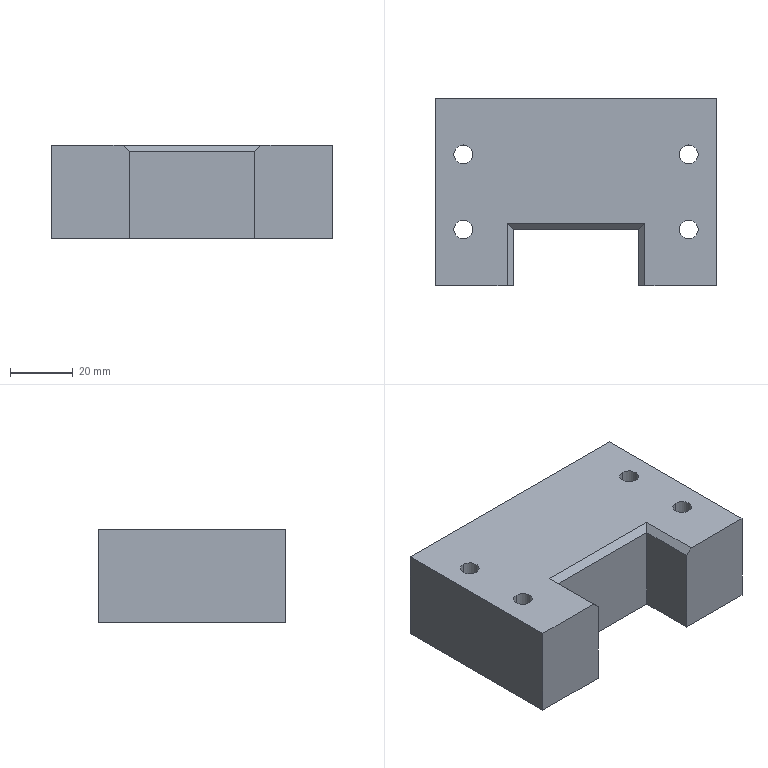Component | SolidWorks | JQ-2-0-006-1 | 1 solid | 29 faces | box 90 x 60 x 30 mm | volume 136495 mm3 | plane 13 | cylinder 12 | cone 4 | commonest cylinder face diameters 6 x8 4.2 x4
build123d program:
from build123d import *

# Parameters (mm, degrees)
SKETCH1_W             = 90
SKETCH1_H             = 30
BOSS_EXTRUDE1_DEPTH   = 60
M5_TAPPED_HOLE1_D     = 4.2
M5_TAPPED_HOLE1_DEPTH = 12.4
M5_TAPPED_HOLE1_TIP   = 1.262
SKETCH5_R             = 3
CUT_EXTRUDE3_DEPTH    = 60
SKETCH6_W             = 40
SKETCH6_H             = 30
CUT_EXTRUDE4_DEPTH    = 18
CHAMFER3_SIZE         = 2


with BuildPart() as part:
    # Sketch1 → Boss-Extrude1 (new body)
    with BuildSketch(Plane.XY):
        with Locations((45, 15)):
            Rectangle(SKETCH1_W, SKETCH1_H)
    extrude(amount=BOSS_EXTRUDE1_DEPTH)

    # M5 Tapped Hole1
    with Locations(Plane(origin=(0, 30, 0), x_dir=(-1, 0, 0), z_dir=(0, 1, 0))):
        with Locations((-25, 30), (-65, 30)):
            Hole(M5_TAPPED_HOLE1_D / 2, depth=M5_TAPPED_HOLE1_DEPTH)
            with Locations((0, 0, -(M5_TAPPED_HOLE1_DEPTH + M5_TAPPED_HOLE1_TIP / 2))):  # 118° drill point
                Cone(0, M5_TAPPED_HOLE1_D / 2, M5_TAPPED_HOLE1_TIP, mode=Mode.SUBTRACT)

    # Sketch5 → Cut-Extrude3 (cut)
    with BuildSketch(Plane(origin=(0, 30, 0), x_dir=(1, 0, 0), z_dir=(0, 1, 0))):
        with Locations(Location((9, -42, 0), (0, 0, 270))):
            Circle(SKETCH5_R)
        with Locations(Location((81, -42, 0), (0, 0, 270))):
            Circle(SKETCH5_R)
        with Locations(Location((81, -18, 0), (0, 0, 270))):
            Circle(SKETCH5_R)
        with Locations(Location((9, -18, 0), (0, 0, 270))):
            Circle(SKETCH5_R)
    extrude(amount=-CUT_EXTRUDE3_DEPTH, mode=Mode.SUBTRACT)

    # Sketch6 → Cut-Extrude4 (cut)
    with BuildSketch(Plane(origin=(0, 0, 0), x_dir=(-1, 0, 0), z_dir=(0, 0, -1))):
        with Locations((-45, 15)):
            Rectangle(SKETCH6_W, SKETCH6_H)
    extrude(amount=-CUT_EXTRUDE4_DEPTH, mode=Mode.SUBTRACT)

    # Chamfer3
    chamfer3_edges = [part.edges().sort_by_distance(p)[0] for p in [
        (45, 0, 18),
        (25, 0, 9),
        (65, 0, 9),
    ]]
    chamfer(chamfer3_edges, length=CHAMFER3_SIZE)


solid = part.part

# Placed as in the assembly
solid = solid.moved(Location((-307.058, -0.6609, 14.131), (-90, 0, 0)))
STEP:
#1=COLOUR_RGB('',0.7922,0.8196,0.9333);
#2=FILL_AREA_STYLE_COLOUR('',#1);
#3=FILL_AREA_STYLE('',(#2));
#4=SURFACE_STYLE_FILL_AREA(#3);
#5=SURFACE_SIDE_STYLE('',(#4));
#6=SURFACE_STYLE_USAGE(.BOTH.,#5);
#7=PRESENTATION_STYLE_ASSIGNMENT((#6));
#8=CARTESIAN_POINT('',(-11.735,0.5645,0.5563));
#9=VERTEX_POINT('',#8);
#10=CARTESIAN_POINT('',(-11.735,0.8008,0.5563));
#11=VERTEX_POINT('',#10);
#12=CARTESIAN_POINT('',(-11.735,0.6826,0.5563));
#13=DIRECTION('',(-0.,0.,-1.));
#14=DIRECTION('',(0.,1.,0.));
#15=AXIS2_PLACEMENT_3D('',#12,#13,#14);
#16=CIRCLE('',#15,0.1181);
#17=EDGE_CURVE('',#9,#11,#16,.T.);
#18=ORIENTED_EDGE('',*,*,#17,.F.);
#19=CARTESIAN_POINT('',(-11.735,0.5645,-0.6248));
#20=VERTEX_POINT('',#19);
#21=CARTESIAN_POINT('',(-11.735,0.5645,1.737));
#22=DIRECTION('',(-0.,0.,-1.));
#23=VECTOR('',#22,39.37);
#24=LINE('',#21,#23);
#25=EDGE_CURVE('',#9,#20,#24,.T.);
#26=ORIENTED_EDGE('',*,*,#25,.T.);
#27=CARTESIAN_POINT('',(-11.735,0.8008,-0.6248));
#28=VERTEX_POINT('',#27);
#29=CARTESIAN_POINT('',(-11.735,0.6826,-0.6248));
#30=DIRECTION('',(-0.,0.,-1.));
#31=DIRECTION('',(0.,1.,0.));
#32=AXIS2_PLACEMENT_3D('',#29,#30,#31);
#33=CIRCLE('',#32,0.1181);
#34=EDGE_CURVE('',#20,#28,#33,.T.);
#35=ORIENTED_EDGE('',*,*,#34,.T.);
#36=CARTESIAN_POINT('',(-11.735,0.8008,1.737));
#37=DIRECTION('',(-0.,0.,-1.));
#38=VECTOR('',#37,39.37);
#39=LINE('',#36,#38);
#40=EDGE_CURVE('',#11,#28,#39,.T.);
#41=ORIENTED_EDGE('',*,*,#40,.F.);
#42=EDGE_LOOP('',(#18,#26,#35,#41));
#43=FACE_OUTER_BOUND('',#42,.T.);
#44=CARTESIAN_POINT('',(-11.735,0.6826,1.737));
#45=DIRECTION('',(-0.,0.,-1.));
#46=DIRECTION('',(0.,1.,0.));
#47=AXIS2_PLACEMENT_3D('',#44,#45,#46);
#48=CYLINDRICAL_SURFACE('',#47,0.1181);
#49=ADVANCED_FACE('',(#43),#48,.F.);
#50=CARTESIAN_POINT('',(-8.9,0.5645,0.5563));
#51=VERTEX_POINT('',#50);
#52=CARTESIAN_POINT('',(-8.9,0.8008,0.5563));
#53=VERTEX_POINT('',#52);
#54=CARTESIAN_POINT('',(-8.9,0.6826,0.5563));
#55=DIRECTION('',(-0.,0.,-1.));
#56=DIRECTION('',(0.,1.,0.));
#57=AXIS2_PLACEMENT_3D('',#54,#55,#56);
#58=CIRCLE('',#57,0.1181);
#59=EDGE_CURVE('',#51,#53,#58,.T.);
#60=ORIENTED_EDGE('',*,*,#59,.F.);
#61=CARTESIAN_POINT('',(-8.9,0.5645,-0.6248));
#62=VERTEX_POINT('',#61);
#63=CARTESIAN_POINT('',(-8.9,0.5645,1.737));
#64=DIRECTION('',(-0.,0.,-1.));
#65=VECTOR('',#64,39.37);
#66=LINE('',#63,#65);
#67=EDGE_CURVE('',#51,#62,#66,.T.);
#68=ORIENTED_EDGE('',*,*,#67,.T.);
#69=CARTESIAN_POINT('',(-8.9,0.8008,-0.6248));
#70=VERTEX_POINT('',#69);
#71=CARTESIAN_POINT('',(-8.9,0.6826,-0.6248));
#72=DIRECTION('',(-0.,0.,-1.));
#73=DIRECTION('',(0.,1.,0.));
#74=AXIS2_PLACEMENT_3D('',#71,#72,#73);
#75=CIRCLE('',#74,0.1181);
#76=EDGE_CURVE('',#62,#70,#75,.T.);
#77=ORIENTED_EDGE('',*,*,#76,.T.);
#78=CARTESIAN_POINT('',(-8.9,0.8008,1.737));
#79=DIRECTION('',(-0.,0.,-1.));
#80=VECTOR('',#79,39.37);
#81=LINE('',#78,#80);
#82=EDGE_CURVE('',#53,#70,#81,.T.);
#83=ORIENTED_EDGE('',*,*,#82,.F.);
#84=EDGE_LOOP('',(#60,#68,#77,#83));
#85=FACE_OUTER_BOUND('',#84,.T.);
#86=CARTESIAN_POINT('',(-8.9,0.6826,1.737));
#87=DIRECTION('',(-0.,0.,-1.));
#88=DIRECTION('',(0.,1.,0.));
#89=AXIS2_PLACEMENT_3D('',#86,#87,#88);
#90=CYLINDRICAL_SURFACE('',#89,0.1181);
#91=ADVANCED_FACE('',(#85),#90,.F.);
#92=CARTESIAN_POINT('',(-8.9,1.509,0.5563));
#93=VERTEX_POINT('',#92);
#94=CARTESIAN_POINT('',(-8.9,1.746,0.5563));
#95=VERTEX_POINT('',#94);
#96=CARTESIAN_POINT('',(-8.9,1.628,0.5563));
#97=DIRECTION('',(-0.,0.,-1.));
#98=DIRECTION('',(0.,1.,0.));
#99=AXIS2_PLACEMENT_3D('',#96,#97,#98);
#100=CIRCLE('',#99,0.1181);
#101=EDGE_CURVE('',#93,#95,#100,.T.);
#102=ORIENTED_EDGE('',*,*,#101,.F.);
#103=CARTESIAN_POINT('',(-8.9,1.509,-0.6248));
#104=VERTEX_POINT('',#103);
#105=CARTESIAN_POINT('',(-8.9,1.509,1.737));
#106=DIRECTION('',(-0.,0.,-1.));
#107=VECTOR('',#106,39.37);
#108=LINE('',#105,#107);
#109=EDGE_CURVE('',#93,#104,#108,.T.);
#110=ORIENTED_EDGE('',*,*,#109,.T.);
#111=CARTESIAN_POINT('',(-8.9,1.746,-0.6248));
#112=VERTEX_POINT('',#111);
#113=CARTESIAN_POINT('',(-8.9,1.628,-0.6248));
#114=DIRECTION('',(-0.,0.,-1.));
#115=DIRECTION('',(0.,1.,0.));
#116=AXIS2_PLACEMENT_3D('',#113,#114,#115);
#117=CIRCLE('',#116,0.1181);
#118=EDGE_CURVE('',#104,#112,#117,.T.);
#119=ORIENTED_EDGE('',*,*,#118,.T.);
#120=CARTESIAN_POINT('',(-8.9,1.746,1.737));
#121=DIRECTION('',(-0.,0.,-1.));
#122=VECTOR('',#121,39.37);
#123=LINE('',#120,#122);
#124=EDGE_CURVE('',#95,#112,#123,.T.);
#125=ORIENTED_EDGE('',*,*,#124,.F.);
#126=EDGE_LOOP('',(#102,#110,#119,#125));
#127=FACE_OUTER_BOUND('',#126,.T.);
#128=CARTESIAN_POINT('',(-8.9,1.628,1.737));
#129=DIRECTION('',(-0.,0.,-1.));
#130=DIRECTION('',(0.,1.,0.));
#131=AXIS2_PLACEMENT_3D('',#128,#129,#130);
#132=CYLINDRICAL_SURFACE('',#131,0.1181);
#133=ADVANCED_FACE('',(#127),#132,.F.);
#134=CARTESIAN_POINT('',(-11.735,1.509,0.5563));
#135=VERTEX_POINT('',#134);
#136=CARTESIAN_POINT('',(-11.735,1.746,0.5563));
#137=VERTEX_POINT('',#136);
#138=CARTESIAN_POINT('',(-11.735,1.628,0.5563));
#139=DIRECTION('',(-0.,0.,-1.));
#140=DIRECTION('',(0.,1.,0.));
#141=AXIS2_PLACEMENT_3D('',#138,#139,#140);
#142=CIRCLE('',#141,0.1181);
#143=EDGE_CURVE('',#135,#137,#142,.T.);
#144=ORIENTED_EDGE('',*,*,#143,.F.);
#145=CARTESIAN_POINT('',(-11.735,1.509,-0.6248));
#146=VERTEX_POINT('',#145);
#147=CARTESIAN_POINT('',(-11.735,1.509,1.737));
#148=DIRECTION('',(-0.,0.,-1.));
#149=VECTOR('',#148,39.37);
#150=LINE('',#147,#149);
#151=EDGE_CURVE('',#135,#146,#150,.T.);
#152=ORIENTED_EDGE('',*,*,#151,.T.);
#153=CARTESIAN_POINT('',(-11.735,1.746,-0.6248));
#154=VERTEX_POINT('',#153);
#155=CARTESIAN_POINT('',(-11.735,1.628,-0.6248));
#156=DIRECTION('',(-0.,0.,-1.));
#157=DIRECTION('',(0.,1.,0.));
#158=AXIS2_PLACEMENT_3D('',#155,#156,#157);
#159=CIRCLE('',#158,0.1181);
#160=EDGE_CURVE('',#146,#154,#159,.T.);
#161=ORIENTED_EDGE('',*,*,#160,.T.);
#162=CARTESIAN_POINT('',(-11.735,1.746,1.737));
#163=DIRECTION('',(-0.,0.,-1.));
#164=VECTOR('',#163,39.37);
#165=LINE('',#162,#164);
#166=EDGE_CURVE('',#137,#154,#165,.T.);
#167=ORIENTED_EDGE('',*,*,#166,.F.);
#168=EDGE_LOOP('',(#144,#152,#161,#167));
#169=FACE_OUTER_BOUND('',#168,.T.);
#170=CARTESIAN_POINT('',(-11.735,1.628,1.737));
#171=DIRECTION('',(-0.,0.,-1.));
#172=DIRECTION('',(0.,1.,0.));
#173=AXIS2_PLACEMENT_3D('',#170,#171,#172);
#174=CYLINDRICAL_SURFACE('',#173,0.1181);
#175=ADVANCED_FACE('',(#169),#174,.F.);
#176=CARTESIAN_POINT('',(-11.105,1.072,-0.1366));
#177=VERTEX_POINT('',#176);
#178=CARTESIAN_POINT('',(-11.105,1.238,-0.1366));
#179=VERTEX_POINT('',#178);
#180=CARTESIAN_POINT('',(-11.105,1.155,-0.1366));
#181=DIRECTION('',(-0.,0.,-1.));
#182=DIRECTION('',(0.,1.,0.));
#183=AXIS2_PLACEMENT_3D('',#180,#181,#182);
#184=CIRCLE('',#183,0.08268);
#185=EDGE_CURVE('',#177,#179,#184,.T.);
#186=ORIENTED_EDGE('',*,*,#185,.F.);
#187=CARTESIAN_POINT('',(-11.105,1.072,-0.6248));
#188=VERTEX_POINT('',#187);
#189=CARTESIAN_POINT('',(-11.105,1.072,-0.6248));
#190=DIRECTION('',(-0.,0.,-1.));
#191=VECTOR('',#190,39.37);
#192=LINE('',#189,#191);
#193=EDGE_CURVE('',#177,#188,#192,.T.);
#194=ORIENTED_EDGE('',*,*,#193,.T.);
#195=CARTESIAN_POINT('',(-11.105,1.238,-0.6248));
#196=VERTEX_POINT('',#195);
#197=CARTESIAN_POINT('',(-11.105,1.155,-0.6248));
#198=DIRECTION('',(-0.,0.,-1.));
#199=DIRECTION('',(0.,1.,0.));
#200=AXIS2_PLACEMENT_3D('',#197,#198,#199);
#201=CIRCLE('',#200,0.08268);
#202=EDGE_CURVE('',#188,#196,#201,.T.);
#203=ORIENTED_EDGE('',*,*,#202,.T.);
#204=CARTESIAN_POINT('',(-11.105,1.238,-0.6248));
#205=DIRECTION('',(-0.,0.,-1.));
#206=VECTOR('',#205,39.37);
#207=LINE('',#204,#206);
#208=EDGE_CURVE('',#179,#196,#207,.T.);
#209=ORIENTED_EDGE('',*,*,#208,.F.);
#210=EDGE_LOOP('',(#186,#194,#203,#209));
#211=FACE_OUTER_BOUND('',#210,.T.);
#212=CARTESIAN_POINT('',(-11.105,1.155,-0.6248));
#213=DIRECTION('',(-0.,0.,-1.));
#214=DIRECTION('',(0.,1.,0.));
#215=AXIS2_PLACEMENT_3D('',#212,#213,#214);
#216=CYLINDRICAL_SURFACE('',#215,0.08268);
#217=ADVANCED_FACE('',(#211),#216,.F.);
#218=CARTESIAN_POINT('',(-11.105,1.155,-0.0869));
#219=VERTEX_POINT('',#218);
#220=CARTESIAN_POINT('',(-11.105,1.238,-0.1366));
#221=DIRECTION('',(0.,0.8572,-0.515));
#222=VECTOR('',#221,39.37);
#223=LINE('',#220,#222);
#224=EDGE_CURVE('',#219,#179,#223,.T.);
#225=ORIENTED_EDGE('',*,*,#224,.F.);
#226=CARTESIAN_POINT('',(-11.105,1.072,-0.1366));
#227=DIRECTION('',(-0.,-0.8572,-0.515));
#228=VECTOR('',#227,39.37);
#229=LINE('',#226,#228);
#230=EDGE_CURVE('',#219,#177,#229,.T.);
#231=ORIENTED_EDGE('',*,*,#230,.T.);
#232=ORIENTED_EDGE('',*,*,#185,.T.);
#233=EDGE_LOOP('',(#225,#231,#232));
#234=FACE_OUTER_BOUND('',#233,.T.);
#235=CARTESIAN_POINT('',(-11.105,1.155,-0.1366));
#236=DIRECTION('',(-0.,0.,-1.));
#237=DIRECTION('',(0.,1.,0.));
#238=AXIS2_PLACEMENT_3D('',#235,#236,#237);
#239=CONICAL_SURFACE('',#238,0.08268,1.03);
#240=ADVANCED_FACE('',(#234),#239,.F.);
#241=CARTESIAN_POINT('',(-9.53,1.072,-0.1366));
#242=VERTEX_POINT('',#241);
#243=CARTESIAN_POINT('',(-9.53,1.238,-0.1366));
#244=VERTEX_POINT('',#243);
#245=CARTESIAN_POINT('',(-9.53,1.155,-0.1366));
#246=DIRECTION('',(-0.,0.,-1.));
#247=DIRECTION('',(0.,1.,0.));
#248=AXIS2_PLACEMENT_3D('',#245,#246,#247);
#249=CIRCLE('',#248,0.08268);
#250=EDGE_CURVE('',#242,#244,#249,.T.);
#251=ORIENTED_EDGE('',*,*,#250,.F.);
#252=CARTESIAN_POINT('',(-9.53,1.072,-0.6248));
#253=VERTEX_POINT('',#252);
#254=CARTESIAN_POINT('',(-9.53,1.072,-0.6248));
#255=DIRECTION('',(-0.,0.,-1.));
#256=VECTOR('',#255,39.37);
#257=LINE('',#254,#256);
#258=EDGE_CURVE('',#242,#253,#257,.T.);
#259=ORIENTED_EDGE('',*,*,#258,.T.);
#260=CARTESIAN_POINT('',(-9.53,1.238,-0.6248));
#261=VERTEX_POINT('',#260);
#262=CARTESIAN_POINT('',(-9.53,1.155,-0.6248));
#263=DIRECTION('',(-0.,0.,-1.));
#264=DIRECTION('',(0.,1.,0.));
#265=AXIS2_PLACEMENT_3D('',#262,#263,#264);
#266=CIRCLE('',#265,0.08268);
#267=EDGE_CURVE('',#253,#261,#266,.T.);
#268=ORIENTED_EDGE('',*,*,#267,.T.);
#269=CARTESIAN_POINT('',(-9.53,1.238,-0.6248));
#270=DIRECTION('',(-0.,0.,-1.));
#271=VECTOR('',#270,39.37);
#272=LINE('',#269,#271);
#273=EDGE_CURVE('',#244,#261,#272,.T.);
#274=ORIENTED_EDGE('',*,*,#273,.F.);
#275=EDGE_LOOP('',(#251,#259,#268,#274));
#276=FACE_OUTER_BOUND('',#275,.T.);
#277=CARTESIAN_POINT('',(-9.53,1.155,-0.6248));
#278=DIRECTION('',(-0.,0.,-1.));
#279=DIRECTION('',(0.,1.,0.));
#280=AXIS2_PLACEMENT_3D('',#277,#278,#279);
#281=CYLINDRICAL_SURFACE('',#280,0.08268);
#282=ADVANCED_FACE('',(#276),#281,.F.);
#283=CARTESIAN_POINT('',(-9.53,1.155,-0.0869));
#284=VERTEX_POINT('',#283);
#285=CARTESIAN_POINT('',(-9.53,1.238,-0.1366));
#286=DIRECTION('',(0.,0.8572,-0.515));
#287=VECTOR('',#286,39.37);
#288=LINE('',#285,#287);
#289=EDGE_CURVE('',#284,#244,#288,.T.);
#290=ORIENTED_EDGE('',*,*,#289,.F.);
#291=CARTESIAN_POINT('',(-9.53,1.072,-0.1366));
#292=DIRECTION('',(-0.,-0.8572,-0.515));
#293=VECTOR('',#292,39.37);
#294=LINE('',#291,#293);
#295=EDGE_CURVE('',#284,#242,#294,.T.);
#296=ORIENTED_EDGE('',*,*,#295,.T.);
#297=ORIENTED_EDGE('',*,*,#250,.T.);
#298=EDGE_LOOP('',(#290,#296,#297));
#299=FACE_OUTER_BOUND('',#298,.T.);
#300=CARTESIAN_POINT('',(-9.53,1.155,-0.1366));
#301=DIRECTION('',(-0.,0.,-1.));
#302=DIRECTION('',(0.,1.,0.));
#303=AXIS2_PLACEMENT_3D('',#300,#301,#302);
#304=CONICAL_SURFACE('',#303,0.08268,1.03);
#305=ADVANCED_FACE('',(#299),#304,.F.);
#306=CARTESIAN_POINT('',(-11.105,-0.02602,0.4776));
#307=VERTEX_POINT('',#306);
#308=CARTESIAN_POINT('',(-11.105,-0.02602,-0.6248));
#309=VERTEX_POINT('',#308);
#310=CARTESIAN_POINT('',(-11.105,-0.02602,0.5563));
#311=DIRECTION('',(-0.,0.,-1.));
#312=VECTOR('',#311,39.37);
#313=LINE('',#310,#312);
#314=EDGE_CURVE('',#307,#309,#313,.T.);
#315=ORIENTED_EDGE('',*,*,#314,.F.);
#316=CARTESIAN_POINT('',(-11.183,-0.02602,0.5563));
#317=VERTEX_POINT('',#316);
#318=CARTESIAN_POINT('',(-11.046,-0.02602,0.4185));
#319=DIRECTION('',(-0.7071,0.,0.7071));
#320=VECTOR('',#319,39.37);
#321=LINE('',#318,#320);
#322=EDGE_CURVE('',#307,#317,#321,.T.);
#323=ORIENTED_EDGE('',*,*,#322,.T.);
#324=CARTESIAN_POINT('',(-12.089,-0.02602,0.5563));
#325=VERTEX_POINT('',#324);
#326=CARTESIAN_POINT('',(-12.089,-0.02602,0.5563));
#327=DIRECTION('',(1.,-0.,-0.));
#328=VECTOR('',#327,39.37);
#329=LINE('',#326,#328);
#330=EDGE_CURVE('',#325,#317,#329,.T.);
#331=ORIENTED_EDGE('',*,*,#330,.F.);
#332=CARTESIAN_POINT('',(-12.089,-0.02602,-0.6248));
#333=VERTEX_POINT('',#332);
#334=CARTESIAN_POINT('',(-12.089,-0.02602,0.5563));
#335=DIRECTION('',(0.,-0.,1.));
#336=VECTOR('',#335,39.37);
#337=LINE('',#334,#336);
#338=EDGE_CURVE('',#333,#325,#337,.T.);
#339=ORIENTED_EDGE('',*,*,#338,.F.);
#340=CARTESIAN_POINT('',(-12.089,-0.02602,-0.6248));
#341=DIRECTION('',(-1.,0.,0.));
#342=VECTOR('',#341,39.37);
#343=LINE('',#340,#342);
#344=EDGE_CURVE('',#309,#333,#343,.T.);
#345=ORIENTED_EDGE('',*,*,#344,.F.);
#346=EDGE_LOOP('',(#315,#323,#331,#339,#345));
#347=FACE_OUTER_BOUND('',#346,.T.);
#348=CARTESIAN_POINT('',(-12.089,-0.02602,-0.6248));
#349=DIRECTION('',(-0.,-1.,-0.));
#350=DIRECTION('',(-1.,0.,0.));
#351=AXIS2_PLACEMENT_3D('',#348,#349,#350);
#352=PLANE('',#351);
#353=ADVANCED_FACE('',(#347),#352,.T.);
#354=ORIENTED_EDGE('',*,*,#338,.T.);
#355=CARTESIAN_POINT('',(-12.089,2.336,0.5563));
#356=VERTEX_POINT('',#355);
#357=CARTESIAN_POINT('',(-12.089,2.336,0.5563));
#358=DIRECTION('',(-0.,-1.,-0.));
#359=VECTOR('',#358,39.37);
#360=LINE('',#357,#359);
#361=EDGE_CURVE('',#356,#325,#360,.T.);
#362=ORIENTED_EDGE('',*,*,#361,.F.);
#363=CARTESIAN_POINT('',(-12.089,2.336,-0.6248));
#364=VERTEX_POINT('',#363);
#365=CARTESIAN_POINT('',(-12.089,2.336,0.5563));
#366=DIRECTION('',(0.,-0.,1.));
#367=VECTOR('',#366,39.37);
#368=LINE('',#365,#367);
#369=EDGE_CURVE('',#364,#356,#368,.T.);
#370=ORIENTED_EDGE('',*,*,#369,.F.);
#371=CARTESIAN_POINT('',(-12.089,2.336,-0.6248));
#372=DIRECTION('',(-0.,-1.,-0.));
#373=VECTOR('',#372,39.37);
#374=LINE('',#371,#373);
#375=EDGE_CURVE('',#364,#333,#374,.T.);
#376=ORIENTED_EDGE('',*,*,#375,.T.);
#377=EDGE_LOOP('',(#354,#362,#370,#376));
#378=FACE_OUTER_BOUND('',#377,.T.);
#379=CARTESIAN_POINT('',(-12.089,2.336,0.5563));
#380=DIRECTION('',(1.,-0.,-0.));
#381=DIRECTION('',(-0.,-1.,-0.));
#382=AXIS2_PLACEMENT_3D('',#379,#380,#381);
#383=PLANE('',#382);
#384=ADVANCED_FACE('',(#378),#383,.F.);
#385=CARTESIAN_POINT('',(-11.183,0.7614,0.5563));
#386=VERTEX_POINT('',#385);
#387=CARTESIAN_POINT('',(-9.451,0.7614,0.5563));
#388=VERTEX_POINT('',#387);
#389=CARTESIAN_POINT('',(-9.53,0.7614,0.5563));
#390=DIRECTION('',(1.,-0.,-0.));
#391=VECTOR('',#390,39.37);
#392=LINE('',#389,#391);
#393=EDGE_CURVE('',#386,#388,#392,.T.);
#394=ORIENTED_EDGE('',*,*,#393,.T.);
#395=CARTESIAN_POINT('',(-9.451,-0.02602,0.5563));
#396=VERTEX_POINT('',#395);
#397=CARTESIAN_POINT('',(-9.451,2.336,0.5563));
#398=DIRECTION('',(-0.,-1.,-0.));
#399=VECTOR('',#398,39.37);
#400=LINE('',#397,#399);
#401=EDGE_CURVE('',#388,#396,#400,.T.);
#402=ORIENTED_EDGE('',*,*,#401,.T.);
#403=CARTESIAN_POINT('',(-8.546,-0.02602,0.5563));
#404=VERTEX_POINT('',#403);
#405=CARTESIAN_POINT('',(-12.089,-0.02602,0.5563));
#406=DIRECTION('',(1.,-0.,-0.));
#407=VECTOR('',#406,39.37);
#408=LINE('',#405,#407);
#409=EDGE_CURVE('',#396,#404,#408,.T.);
#410=ORIENTED_EDGE('',*,*,#409,.T.);
#411=CARTESIAN_POINT('',(-8.546,2.336,0.5563));
#412=VERTEX_POINT('',#411);
#413=CARTESIAN_POINT('',(-8.546,2.336,0.5563));
#414=DIRECTION('',(-0.,-1.,-0.));
#415=VECTOR('',#414,39.37);
#416=LINE('',#413,#415);
#417=EDGE_CURVE('',#412,#404,#416,.T.);
#418=ORIENTED_EDGE('',*,*,#417,.F.);
#419=CARTESIAN_POINT('',(-12.089,2.336,0.5563));
#420=DIRECTION('',(1.,-0.,-0.));
#421=VECTOR('',#420,39.37);
#422=LINE('',#419,#421);
#423=EDGE_CURVE('',#356,#412,#422,.T.);
#424=ORIENTED_EDGE('',*,*,#423,.F.);
#425=ORIENTED_EDGE('',*,*,#361,.T.);
#426=ORIENTED_EDGE('',*,*,#330,.T.);
#427=CARTESIAN_POINT('',(-11.183,2.336,0.5563));
#428=DIRECTION('',(0.,1.,0.));
#429=VECTOR('',#428,39.37);
#430=LINE('',#427,#429);
#431=EDGE_CURVE('',#317,#386,#430,.T.);
#432=ORIENTED_EDGE('',*,*,#431,.T.);
#433=EDGE_LOOP('',(#394,#402,#410,#418,#424,#425,#426,#432));
#434=FACE_OUTER_BOUND('',#433,.T.);
#435=CARTESIAN_POINT('',(-11.735,0.6826,0.5563));
#436=DIRECTION('',(-0.,0.,-1.));
#437=DIRECTION('',(0.,1.,0.));
#438=AXIS2_PLACEMENT_3D('',#435,#436,#437);
#439=CIRCLE('',#438,0.1181);
#440=EDGE_CURVE('',#11,#9,#439,.T.);
#441=ORIENTED_EDGE('',*,*,#440,.T.);
#442=ORIENTED_EDGE('',*,*,#17,.T.);
#443=EDGE_LOOP('',(#441,#442));
#444=FACE_BOUND('',#443,.T.);
#445=CARTESIAN_POINT('',(-8.9,0.6826,0.5563));
#446=DIRECTION('',(-0.,0.,-1.));
#447=DIRECTION('',(0.,1.,0.));
#448=AXIS2_PLACEMENT_3D('',#445,#446,#447);
#449=CIRCLE('',#448,0.1181);
#450=EDGE_CURVE('',#53,#51,#449,.T.);
#451=ORIENTED_EDGE('',*,*,#450,.T.);
#452=ORIENTED_EDGE('',*,*,#59,.T.);
#453=EDGE_LOOP('',(#451,#452));
#454=FACE_BOUND('',#453,.T.);
#455=CARTESIAN_POINT('',(-8.9,1.628,0.5563));
#456=DIRECTION('',(-0.,0.,-1.));
#457=DIRECTION('',(0.,1.,0.));
#458=AXIS2_PLACEMENT_3D('',#455,#456,#457);
#459=CIRCLE('',#458,0.1181);
#460=EDGE_CURVE('',#95,#93,#459,.T.);
#461=ORIENTED_EDGE('',*,*,#460,.T.);
#462=ORIENTED_EDGE('',*,*,#101,.T.);
#463=EDGE_LOOP('',(#461,#462));
#464=FACE_BOUND('',#463,.T.);
#465=CARTESIAN_POINT('',(-11.735,1.628,0.5563));
#466=DIRECTION('',(-0.,0.,-1.));
#467=DIRECTION('',(0.,1.,0.));
#468=AXIS2_PLACEMENT_3D('',#465,#466,#467);
#469=CIRCLE('',#468,0.1181);
#470=EDGE_CURVE('',#137,#135,#469,.T.);
#471=ORIENTED_EDGE('',*,*,#470,.T.);
#472=ORIENTED_EDGE('',*,*,#143,.T.);
#473=EDGE_LOOP('',(#471,#472));
#474=FACE_BOUND('',#473,.T.);
#475=CARTESIAN_POINT('',(-12.089,2.336,0.5563));
#476=DIRECTION('',(-0.,0.,-1.));
#477=DIRECTION('',(0.,1.,0.));
#478=AXIS2_PLACEMENT_3D('',#475,#476,#477);
#479=PLANE('',#478);
#480=ADVANCED_FACE('',(#434,#444,#454,#464,#474),#479,.F.);
#481=CARTESIAN_POINT('',(-8.546,-0.02602,-0.6248));
#482=VERTEX_POINT('',#481);
#483=CARTESIAN_POINT('',(-8.546,-0.02602,0.5563));
#484=DIRECTION('',(-0.,0.,-1.));
#485=VECTOR('',#484,39.37);
#486=LINE('',#483,#485);
#487=EDGE_CURVE('',#404,#482,#486,.T.);
#488=ORIENTED_EDGE('',*,*,#487,.T.);
#489=CARTESIAN_POINT('',(-8.546,2.336,-0.6248));
#490=VERTEX_POINT('',#489);
#491=CARTESIAN_POINT('',(-8.546,2.336,-0.6248));
#492=DIRECTION('',(-0.,-1.,-0.));
#493=VECTOR('',#492,39.37);
#494=LINE('',#491,#493);
#495=EDGE_CURVE('',#490,#482,#494,.T.);
#496=ORIENTED_EDGE('',*,*,#495,.F.);
#497=CARTESIAN_POINT('',(-8.546,2.336,0.5563));
#498=DIRECTION('',(-0.,0.,-1.));
#499=VECTOR('',#498,39.37);
#500=LINE('',#497,#499);
#501=EDGE_CURVE('',#412,#490,#500,.T.);
#502=ORIENTED_EDGE('',*,*,#501,.F.);
#503=ORIENTED_EDGE('',*,*,#417,.T.);
#504=EDGE_LOOP('',(#488,#496,#502,#503));
#505=FACE_OUTER_BOUND('',#504,.T.);
#506=CARTESIAN_POINT('',(-8.546,2.336,0.5563));
#507=DIRECTION('',(-1.,0.,0.));
#508=DIRECTION('',(0.,1.,0.));
#509=AXIS2_PLACEMENT_3D('',#506,#507,#508);
#510=PLANE('',#509);
#511=ADVANCED_FACE('',(#505),#510,.F.);
#512=CARTESIAN_POINT('',(-11.735,0.6826,-0.6248));
#513=DIRECTION('',(-0.,0.,-1.));
#514=DIRECTION('',(0.,1.,0.));
#515=AXIS2_PLACEMENT_3D('',#512,#513,#514);
#516=CIRCLE('',#515,0.1181);
#517=EDGE_CURVE('',#28,#20,#516,.T.);
#518=ORIENTED_EDGE('',*,*,#517,.F.);
#519=ORIENTED_EDGE('',*,*,#34,.F.);
#520=EDGE_LOOP('',(#518,#519));
#521=FACE_BOUND('',#520,.T.);
#522=CARTESIAN_POINT('',(-8.9,0.6826,-0.6248));
#523=DIRECTION('',(-0.,0.,-1.));
#524=DIRECTION('',(0.,1.,0.));
#525=AXIS2_PLACEMENT_3D('',#522,#523,#524);
#526=CIRCLE('',#525,0.1181);
#527=EDGE_CURVE('',#70,#62,#526,.T.);
#528=ORIENTED_EDGE('',*,*,#527,.F.);
#529=ORIENTED_EDGE('',*,*,#76,.F.);
#530=EDGE_LOOP('',(#528,#529));
#531=FACE_BOUND('',#530,.T.);
#532=CARTESIAN_POINT('',(-8.9,1.628,-0.6248));
#533=DIRECTION('',(-0.,0.,-1.));
#534=DIRECTION('',(0.,1.,0.));
#535=AXIS2_PLACEMENT_3D('',#532,#533,#534);
#536=CIRCLE('',#535,0.1181);
#537=EDGE_CURVE('',#112,#104,#536,.T.);
#538=ORIENTED_EDGE('',*,*,#537,.F.);
#539=ORIENTED_EDGE('',*,*,#118,.F.);
#540=EDGE_LOOP('',(#538,#539));
#541=FACE_BOUND('',#540,.T.);
#542=CARTESIAN_POINT('',(-11.735,1.628,-0.6248));
#543=DIRECTION('',(-0.,0.,-1.));
#544=DIRECTION('',(0.,1.,0.));
#545=AXIS2_PLACEMENT_3D('',#542,#543,#544);
#546=CIRCLE('',#545,0.1181);
#547=EDGE_CURVE('',#154,#146,#546,.T.);
#548=ORIENTED_EDGE('',*,*,#547,.F.);
#549=ORIENTED_EDGE('',*,*,#160,.F.);
#550=EDGE_LOOP('',(#548,#549));
#551=FACE_BOUND('',#550,.T.);
#552=CARTESIAN_POINT('',(-11.105,1.155,-0.6248));
#553=DIRECTION('',(-0.,0.,-1.));
#554=DIRECTION('',(0.,1.,0.));
#555=AXIS2_PLACEMENT_3D('',#552,#553,#554);
#556=CIRCLE('',#555,0.08268);
#557=EDGE_CURVE('',#196,#188,#556,.T.);
#558=ORIENTED_EDGE('',*,*,#557,.F.);
#559=ORIENTED_EDGE('',*,*,#202,.F.);
#560=EDGE_LOOP('',(#558,#559));
#561=FACE_BOUND('',#560,.T.);
#562=CARTESIAN_POINT('',(-9.53,1.155,-0.6248));
#563=DIRECTION('',(-0.,0.,-1.));
#564=DIRECTION('',(0.,1.,0.));
#565=AXIS2_PLACEMENT_3D('',#562,#563,#564);
#566=CIRCLE('',#565,0.08268);
#567=EDGE_CURVE('',#261,#253,#566,.T.);
#568=ORIENTED_EDGE('',*,*,#567,.F.);
#569=ORIENTED_EDGE('',*,*,#267,.F.);
#570=EDGE_LOOP('',(#568,#569));
#571=FACE_BOUND('',#570,.T.);
#572=CARTESIAN_POINT('',(-11.105,0.6826,-0.6248));
#573=VERTEX_POINT('',#572);
#574=CARTESIAN_POINT('',(-9.53,0.6826,-0.6248));
#575=VERTEX_POINT('',#574);
#576=CARTESIAN_POINT('',(-11.105,0.6826,-0.6248));
#577=DIRECTION('',(1.,-0.,-0.));
#578=VECTOR('',#577,39.37);
#579=LINE('',#576,#578);
#580=EDGE_CURVE('',#573,#575,#579,.T.);
#581=ORIENTED_EDGE('',*,*,#580,.F.);
#582=CARTESIAN_POINT('',(-11.105,0.6826,-0.6248));
#583=DIRECTION('',(-0.,-1.,-0.));
#584=VECTOR('',#583,39.37);
#585=LINE('',#582,#584);
#586=EDGE_CURVE('',#573,#309,#585,.T.);
#587=ORIENTED_EDGE('',*,*,#586,.T.);
#588=ORIENTED_EDGE('',*,*,#344,.T.);
#589=ORIENTED_EDGE('',*,*,#375,.F.);
#590=CARTESIAN_POINT('',(-12.089,2.336,-0.6248));
#591=DIRECTION('',(-1.,0.,0.));
#592=VECTOR('',#591,39.37);
#593=LINE('',#590,#592);
#594=EDGE_CURVE('',#490,#364,#593,.T.);
#595=ORIENTED_EDGE('',*,*,#594,.F.);
#596=ORIENTED_EDGE('',*,*,#495,.T.);
#597=CARTESIAN_POINT('',(-9.53,-0.02602,-0.6248));
#598=VERTEX_POINT('',#597);
#599=CARTESIAN_POINT('',(-12.089,-0.02602,-0.6248));
#600=DIRECTION('',(-1.,0.,0.));
#601=VECTOR('',#600,39.37);
#602=LINE('',#599,#601);
#603=EDGE_CURVE('',#482,#598,#602,.T.);
#604=ORIENTED_EDGE('',*,*,#603,.T.);
#605=CARTESIAN_POINT('',(-9.53,0.6826,-0.6248));
#606=DIRECTION('',(-0.,-1.,-0.));
#607=VECTOR('',#606,39.37);
#608=LINE('',#605,#607);
#609=EDGE_CURVE('',#575,#598,#608,.T.);
#610=ORIENTED_EDGE('',*,*,#609,.F.);
#611=EDGE_LOOP('',(#581,#587,#588,#589,#595,#596,#604,#610));
#612=FACE_OUTER_BOUND('',#611,.T.);
#613=CARTESIAN_POINT('',(-12.089,2.336,-0.6248));
#614=DIRECTION('',(0.,-0.,1.));
#615=DIRECTION('',(-0.,-1.,-0.));
#616=AXIS2_PLACEMENT_3D('',#613,#614,#615);
#617=PLANE('',#616);
#618=ADVANCED_FACE('',(#521,#531,#541,#551,#561,#571,#612),#617,.F.);
#619=ORIENTED_EDGE('',*,*,#369,.T.);
#620=ORIENTED_EDGE('',*,*,#423,.T.);
#621=ORIENTED_EDGE('',*,*,#501,.T.);
#622=ORIENTED_EDGE('',*,*,#594,.T.);
#623=EDGE_LOOP('',(#619,#620,#621,#622));
#624=FACE_OUTER_BOUND('',#623,.T.);
#625=CARTESIAN_POINT('',(-12.089,2.336,-0.6248));
#626=DIRECTION('',(-0.,-1.,-0.));
#627=DIRECTION('',(-1.,0.,0.));
#628=AXIS2_PLACEMENT_3D('',#625,#626,#627);
#629=PLANE('',#628);
#630=ADVANCED_FACE('',(#624),#629,.F.);
#631=ORIENTED_EDGE('',*,*,#409,.F.);
#632=CARTESIAN_POINT('',(-9.53,-0.02602,0.4776));
#633=VERTEX_POINT('',#632);
#634=CARTESIAN_POINT('',(-11.361,-0.02602,-1.353));
#635=DIRECTION('',(-0.7071,0.,-0.7071));
#636=VECTOR('',#635,39.37);
#637=LINE('',#634,#636);
#638=EDGE_CURVE('',#396,#633,#637,.T.);
#639=ORIENTED_EDGE('',*,*,#638,.T.);
#640=CARTESIAN_POINT('',(-9.53,-0.02602,0.5563));
#641=DIRECTION('',(0.,-0.,1.));
#642=VECTOR('',#641,39.37);
#643=LINE('',#640,#642);
#644=EDGE_CURVE('',#598,#633,#643,.T.);
#645=ORIENTED_EDGE('',*,*,#644,.F.);
#646=ORIENTED_EDGE('',*,*,#603,.F.);
#647=ORIENTED_EDGE('',*,*,#487,.F.);
#648=EDGE_LOOP('',(#631,#639,#645,#646,#647));
#649=FACE_OUTER_BOUND('',#648,.T.);
#650=CARTESIAN_POINT('',(-12.089,-0.02602,-0.6248));
#651=DIRECTION('',(-0.,-1.,-0.));
#652=DIRECTION('',(-1.,0.,0.));
#653=AXIS2_PLACEMENT_3D('',#650,#651,#652);
#654=PLANE('',#653);
#655=ADVANCED_FACE('',(#649),#654,.T.);
#656=ORIENTED_EDGE('',*,*,#295,.F.);
#657=ORIENTED_EDGE('',*,*,#289,.T.);
#658=CARTESIAN_POINT('',(-9.53,1.155,-0.1366));
#659=DIRECTION('',(-0.,0.,-1.));
#660=DIRECTION('',(0.,1.,0.));
#661=AXIS2_PLACEMENT_3D('',#658,#659,#660);
#662=CIRCLE('',#661,0.08268);
#663=EDGE_CURVE('',#244,#242,#662,.T.);
#664=ORIENTED_EDGE('',*,*,#663,.T.);
#665=EDGE_LOOP('',(#656,#657,#664));
#666=FACE_OUTER_BOUND('',#665,.T.);
#667=CARTESIAN_POINT('',(-9.53,1.155,-0.1366));
#668=DIRECTION('',(-0.,0.,-1.));
#669=DIRECTION('',(0.,1.,0.));
#670=AXIS2_PLACEMENT_3D('',#667,#668,#669);
#671=CONICAL_SURFACE('',#670,0.08268,1.03);
#672=ADVANCED_FACE('',(#666),#671,.F.);
#673=ORIENTED_EDGE('',*,*,#258,.F.);
#674=ORIENTED_EDGE('',*,*,#663,.F.);
#675=ORIENTED_EDGE('',*,*,#273,.T.);
#676=ORIENTED_EDGE('',*,*,#567,.T.);
#677=EDGE_LOOP('',(#673,#674,#675,#676));
#678=FACE_OUTER_BOUND('',#677,.T.);
#679=CARTESIAN_POINT('',(-9.53,1.155,-0.6248));
#680=DIRECTION('',(-0.,0.,-1.));
#681=DIRECTION('',(0.,1.,0.));
#682=AXIS2_PLACEMENT_3D('',#679,#680,#681);
#683=CYLINDRICAL_SURFACE('',#682,0.08268);
#684=ADVANCED_FACE('',(#678),#683,.F.);
#685=ORIENTED_EDGE('',*,*,#230,.F.);
#686=ORIENTED_EDGE('',*,*,#224,.T.);
#687=CARTESIAN_POINT('',(-11.105,1.155,-0.1366));
#688=DIRECTION('',(-0.,0.,-1.));
#689=DIRECTION('',(0.,1.,0.));
#690=AXIS2_PLACEMENT_3D('',#687,#688,#689);
#691=CIRCLE('',#690,0.08268);
#692=EDGE_CURVE('',#179,#177,#691,.T.);
#693=ORIENTED_EDGE('',*,*,#692,.T.);
#694=EDGE_LOOP('',(#685,#686,#693));
#695=FACE_OUTER_BOUND('',#694,.T.);
#696=CARTESIAN_POINT('',(-11.105,1.155,-0.1366));
#697=DIRECTION('',(-0.,0.,-1.));
#698=DIRECTION('',(0.,1.,0.));
#699=AXIS2_PLACEMENT_3D('',#696,#697,#698);
#700=CONICAL_SURFACE('',#699,0.08268,1.03);
#701=ADVANCED_FACE('',(#695),#700,.F.);
#702=ORIENTED_EDGE('',*,*,#193,.F.);
#703=ORIENTED_EDGE('',*,*,#692,.F.);
#704=ORIENTED_EDGE('',*,*,#208,.T.);
#705=ORIENTED_EDGE('',*,*,#557,.T.);
#706=EDGE_LOOP('',(#702,#703,#704,#705));
#707=FACE_OUTER_BOUND('',#706,.T.);
#708=CARTESIAN_POINT('',(-11.105,1.155,-0.6248));
#709=DIRECTION('',(-0.,0.,-1.));
#710=DIRECTION('',(0.,1.,0.));
#711=AXIS2_PLACEMENT_3D('',#708,#709,#710);
#712=CYLINDRICAL_SURFACE('',#711,0.08268);
#713=ADVANCED_FACE('',(#707),#712,.F.);
#714=ORIENTED_EDGE('',*,*,#151,.F.);
#715=ORIENTED_EDGE('',*,*,#470,.F.);
#716=ORIENTED_EDGE('',*,*,#166,.T.);
#717=ORIENTED_EDGE('',*,*,#547,.T.);
#718=EDGE_LOOP('',(#714,#715,#716,#717));
#719=FACE_OUTER_BOUND('',#718,.T.);
#720=CARTESIAN_POINT('',(-11.735,1.628,1.737));
#721=DIRECTION('',(-0.,0.,-1.));
#722=DIRECTION('',(0.,1.,0.));
#723=AXIS2_PLACEMENT_3D('',#720,#721,#722);
#724=CYLINDRICAL_SURFACE('',#723,0.1181);
#725=ADVANCED_FACE('',(#719),#724,.F.);
#726=ORIENTED_EDGE('',*,*,#109,.F.);
#727=ORIENTED_EDGE('',*,*,#460,.F.);
#728=ORIENTED_EDGE('',*,*,#124,.T.);
#729=ORIENTED_EDGE('',*,*,#537,.T.);
#730=EDGE_LOOP('',(#726,#727,#728,#729));
#731=FACE_OUTER_BOUND('',#730,.T.);
#732=CARTESIAN_POINT('',(-8.9,1.628,1.737));
#733=DIRECTION('',(-0.,0.,-1.));
#734=DIRECTION('',(0.,1.,0.));
#735=AXIS2_PLACEMENT_3D('',#732,#733,#734);
#736=CYLINDRICAL_SURFACE('',#735,0.1181);
#737=ADVANCED_FACE('',(#731),#736,.F.);
#738=ORIENTED_EDGE('',*,*,#67,.F.);
#739=ORIENTED_EDGE('',*,*,#450,.F.);
#740=ORIENTED_EDGE('',*,*,#82,.T.);
#741=ORIENTED_EDGE('',*,*,#527,.T.);
#742=EDGE_LOOP('',(#738,#739,#740,#741));
#743=FACE_OUTER_BOUND('',#742,.T.);
#744=CARTESIAN_POINT('',(-8.9,0.6826,1.737));
#745=DIRECTION('',(-0.,0.,-1.));
#746=DIRECTION('',(0.,1.,0.));
#747=AXIS2_PLACEMENT_3D('',#744,#745,#746);
#748=CYLINDRICAL_SURFACE('',#747,0.1181);
#749=ADVANCED_FACE('',(#743),#748,.F.);
#750=ORIENTED_EDGE('',*,*,#25,.F.);
#751=ORIENTED_EDGE('',*,*,#440,.F.);
#752=ORIENTED_EDGE('',*,*,#40,.T.);
#753=ORIENTED_EDGE('',*,*,#517,.T.);
#754=EDGE_LOOP('',(#750,#751,#752,#753));
#755=FACE_OUTER_BOUND('',#754,.T.);
#756=CARTESIAN_POINT('',(-11.735,0.6826,1.737));
#757=DIRECTION('',(-0.,0.,-1.));
#758=DIRECTION('',(0.,1.,0.));
#759=AXIS2_PLACEMENT_3D('',#756,#757,#758);
#760=CYLINDRICAL_SURFACE('',#759,0.1181);
#761=ADVANCED_FACE('',(#755),#760,.F.);
#762=CARTESIAN_POINT('',(-11.105,0.6826,0.4776));
#763=VERTEX_POINT('',#762);
#764=CARTESIAN_POINT('',(-11.105,0.6826,0.5563));
#765=DIRECTION('',(-0.,0.,-1.));
#766=VECTOR('',#765,39.37);
#767=LINE('',#764,#766);
#768=EDGE_CURVE('',#763,#573,#767,.T.);
#769=ORIENTED_EDGE('',*,*,#768,.F.);
#770=CARTESIAN_POINT('',(-11.105,0.6826,0.4776));
#771=DIRECTION('',(-0.,-1.,-0.));
#772=VECTOR('',#771,39.37);
#773=LINE('',#770,#772);
#774=EDGE_CURVE('',#763,#307,#773,.T.);
#775=ORIENTED_EDGE('',*,*,#774,.T.);
#776=ORIENTED_EDGE('',*,*,#314,.T.);
#777=ORIENTED_EDGE('',*,*,#586,.F.);
#778=EDGE_LOOP('',(#769,#775,#776,#777));
#779=FACE_OUTER_BOUND('',#778,.T.);
#780=CARTESIAN_POINT('',(-11.105,0.6826,0.5563));
#781=DIRECTION('',(-1.,0.,0.));
#782=DIRECTION('',(0.,1.,0.));
#783=AXIS2_PLACEMENT_3D('',#780,#781,#782);
#784=PLANE('',#783);
#785=ADVANCED_FACE('',(#779),#784,.F.);
#786=ORIENTED_EDGE('',*,*,#644,.T.);
#787=CARTESIAN_POINT('',(-9.53,0.6826,0.4776));
#788=VERTEX_POINT('',#787);
#789=CARTESIAN_POINT('',(-9.53,0.6826,0.4776));
#790=DIRECTION('',(0.,1.,0.));
#791=VECTOR('',#790,39.37);
#792=LINE('',#789,#791);
#793=EDGE_CURVE('',#633,#788,#792,.T.);
#794=ORIENTED_EDGE('',*,*,#793,.T.);
#795=CARTESIAN_POINT('',(-9.53,0.6826,0.5563));
#796=DIRECTION('',(0.,-0.,1.));
#797=VECTOR('',#796,39.37);
#798=LINE('',#795,#797);
#799=EDGE_CURVE('',#575,#788,#798,.T.);
#800=ORIENTED_EDGE('',*,*,#799,.F.);
#801=ORIENTED_EDGE('',*,*,#609,.T.);
#802=EDGE_LOOP('',(#786,#794,#800,#801));
#803=FACE_OUTER_BOUND('',#802,.T.);
#804=CARTESIAN_POINT('',(-9.53,0.6826,0.5563));
#805=DIRECTION('',(1.,-0.,-0.));
#806=DIRECTION('',(-0.,-1.,-0.));
#807=AXIS2_PLACEMENT_3D('',#804,#805,#806);
#808=PLANE('',#807);
#809=ADVANCED_FACE('',(#803),#808,.F.);
#810=ORIENTED_EDGE('',*,*,#799,.T.);
#811=CARTESIAN_POINT('',(-11.105,0.6826,0.4776));
#812=DIRECTION('',(-1.,0.,0.));
#813=VECTOR('',#812,39.37);
#814=LINE('',#811,#813);
#815=EDGE_CURVE('',#788,#763,#814,.T.);
#816=ORIENTED_EDGE('',*,*,#815,.T.);
#817=ORIENTED_EDGE('',*,*,#768,.T.);
#818=ORIENTED_EDGE('',*,*,#580,.T.);
#819=EDGE_LOOP('',(#810,#816,#817,#818));
#820=FACE_OUTER_BOUND('',#819,.T.);
#821=CARTESIAN_POINT('',(-12.089,0.6826,0.5563));
#822=DIRECTION('',(-0.,-1.,-0.));
#823=DIRECTION('',(-1.,0.,0.));
#824=AXIS2_PLACEMENT_3D('',#821,#822,#823);
#825=PLANE('',#824);
#826=ADVANCED_FACE('',(#820),#825,.T.);
#827=ORIENTED_EDGE('',*,*,#322,.F.);
#828=ORIENTED_EDGE('',*,*,#774,.F.);
#829=CARTESIAN_POINT('',(-11.433,1.011,0.8057));
#830=DIRECTION('',(0.5774,-0.5774,-0.5774));
#831=VECTOR('',#830,39.37);
#832=LINE('',#829,#831);
#833=EDGE_CURVE('',#386,#763,#832,.T.);
#834=ORIENTED_EDGE('',*,*,#833,.F.);
#835=ORIENTED_EDGE('',*,*,#431,.F.);
#836=EDGE_LOOP('',(#827,#828,#834,#835));
#837=FACE_OUTER_BOUND('',#836,.T.);
#838=CARTESIAN_POINT('',(-11.105,0.6826,0.4776));
#839=DIRECTION('',(-0.7071,0.,-0.7071));
#840=DIRECTION('',(-0.,-1.,-0.));
#841=AXIS2_PLACEMENT_3D('',#838,#839,#840);
#842=PLANE('',#841);
#843=ADVANCED_FACE('',(#837),#842,.F.);
#844=ORIENTED_EDGE('',*,*,#833,.T.);
#845=ORIENTED_EDGE('',*,*,#815,.F.);
#846=CARTESIAN_POINT('',(-8.926,1.286,1.081));
#847=DIRECTION('',(-0.5774,-0.5774,-0.5774));
#848=VECTOR('',#847,39.37);
#849=LINE('',#846,#848);
#850=EDGE_CURVE('',#388,#788,#849,.T.);
#851=ORIENTED_EDGE('',*,*,#850,.F.);
#852=ORIENTED_EDGE('',*,*,#393,.F.);
#853=EDGE_LOOP('',(#844,#845,#851,#852));
#854=FACE_OUTER_BOUND('',#853,.T.);
#855=CARTESIAN_POINT('',(-12.089,0.6826,0.4776));
#856=DIRECTION('',(-0.,-0.7071,0.7071));
#857=DIRECTION('',(1.,-0.,-0.));
#858=AXIS2_PLACEMENT_3D('',#855,#856,#857);
#859=PLANE('',#858);
#860=ADVANCED_FACE('',(#854),#859,.T.);
#861=ORIENTED_EDGE('',*,*,#850,.T.);
#862=ORIENTED_EDGE('',*,*,#793,.F.);
#863=ORIENTED_EDGE('',*,*,#638,.F.);
#864=ORIENTED_EDGE('',*,*,#401,.F.);
#865=EDGE_LOOP('',(#861,#862,#863,#864));
#866=FACE_OUTER_BOUND('',#865,.T.);
#867=CARTESIAN_POINT('',(-9.451,2.336,0.5563));
#868=DIRECTION('',(0.7071,-0.,-0.7071));
#869=DIRECTION('',(-0.,-1.,-0.));
#870=AXIS2_PLACEMENT_3D('',#867,#868,#869);
#871=PLANE('',#870);
#872=ADVANCED_FACE('',(#866),#871,.F.);
#873=CLOSED_SHELL('',(#49,#91,#133,#175,#217,#240,#282,#305,#353,#384,#480,#511,#618,#630,#655,#672,#684,#701,#713,#725,#737,#749,#761,#785,#809,#826,#843,#860,#872));
#874=MANIFOLD_SOLID_BREP('',#873);
#875=STYLED_ITEM('',(#7),#874);
#876=PRESENTATION_LAYER_ASSIGNMENT('','',(#875));
#877=CARTESIAN_POINT('',(0.,0.,0.));
#878=DIRECTION('',(0.,0.,1.));
#879=DIRECTION('',(1.,0.,0.));
#880=AXIS2_PLACEMENT_3D('',#877,#878,#879);
#881=(LENGTH_UNIT()NAMED_UNIT(*)SI_UNIT($,.METRE.));
#882=LENGTH_MEASURE_WITH_UNIT(LENGTH_MEASURE(0.0254),#881);
#883=DIMENSIONAL_EXPONENTS(1.,0.,0.,0.,0.,0.,0.);
#884=(CONVERSION_BASED_UNIT('',#882)LENGTH_UNIT()NAMED_UNIT(#883));
#885=UNCERTAINTY_MEASURE_WITH_UNIT(LENGTH_MEASURE(0.00001),#884,'','');
#886=(NAMED_UNIT(*)PLANE_ANGLE_UNIT()SI_UNIT($,.RADIAN.));
#887=(NAMED_UNIT(*)SI_UNIT($,.STERADIAN.)SOLID_ANGLE_UNIT());
#888=(GEOMETRIC_REPRESENTATION_CONTEXT(3)GLOBAL_UNCERTAINTY_ASSIGNED_CONTEXT((#885))GLOBAL_UNIT_ASSIGNED_CONTEXT((#884,#886,#887))REPRESENTATION_CONTEXT('',''));
#889=ADVANCED_BREP_SHAPE_REPRESENTATION('',(#874,#880),#888);
#890=(LENGTH_UNIT()NAMED_UNIT(*)SI_UNIT($,.METRE.));
#891=LENGTH_MEASURE_WITH_UNIT(LENGTH_MEASURE(0.0254),#890);
#892=DIMENSIONAL_EXPONENTS(1.,0.,0.,0.,0.,0.,0.);
#893=(CONVERSION_BASED_UNIT('',#891)LENGTH_UNIT()NAMED_UNIT(#892));
#894=UNCERTAINTY_MEASURE_WITH_UNIT(LENGTH_MEASURE(0.00001),#893,'','');
#895=(NAMED_UNIT(*)PLANE_ANGLE_UNIT()SI_UNIT($,.RADIAN.));
#896=(NAMED_UNIT(*)SI_UNIT($,.STERADIAN.)SOLID_ANGLE_UNIT());
#897=(GEOMETRIC_REPRESENTATION_CONTEXT(3)GLOBAL_UNCERTAINTY_ASSIGNED_CONTEXT((#894))GLOBAL_UNIT_ASSIGNED_CONTEXT((#893,#895,#896))REPRESENTATION_CONTEXT('',''));
#898=MECHANICAL_DESIGN_GEOMETRIC_PRESENTATION_REPRESENTATION('',(#875),#897);